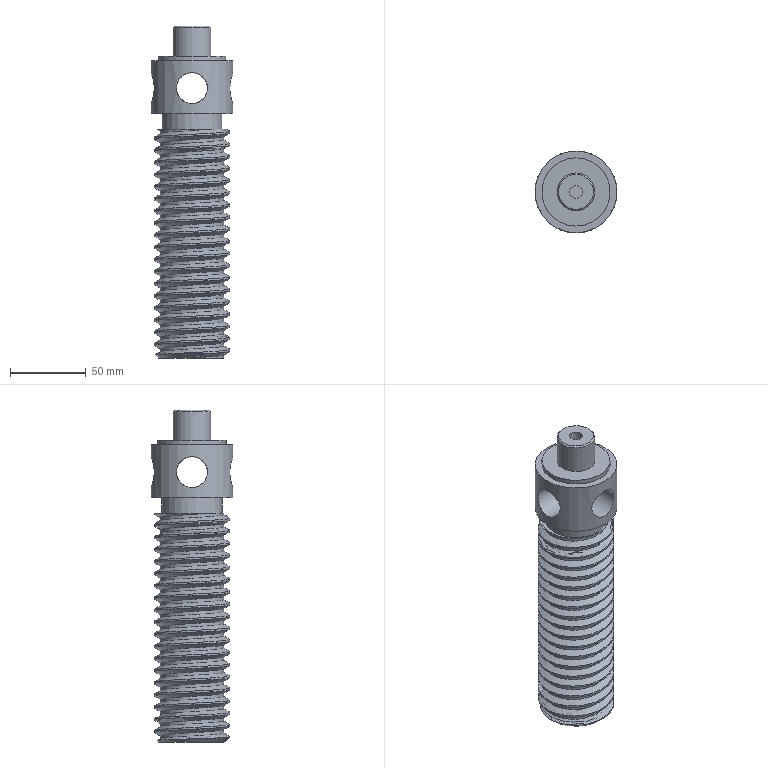Component | NX | LEAD_SCREW | 1 solid | 22 faces | volume 323968 mm3 | cylinder 11 | plane 7 | cone 2 | spline 2 | commonest cylinder face diameters 20.5 x4 50 x1 25 x1 45 x1 54 x1 40 x1 8.5 x1 42 x1